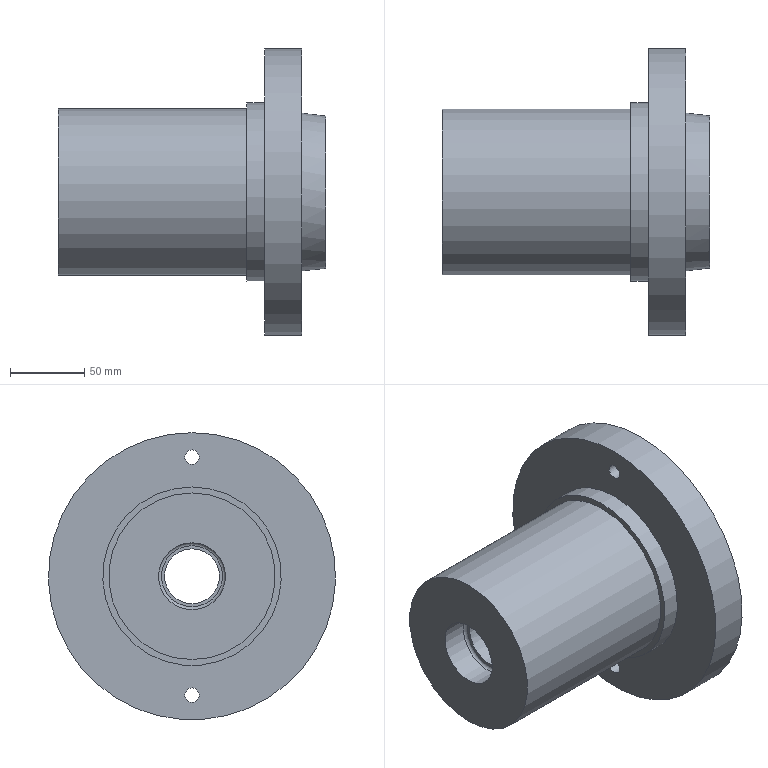Component | NX | CA614_SPINDLE | 1 solid | 16 faces | box 179.52 x 193 x 193 mm | volume 1954498 mm3 | cylinder 6 | plane 6 | cone 3 | torus 1 | commonest cylinder face diameters 9.732 x2 193 x1 45 x1 112 x1 120 x1
STEP:
#1=CARTESIAN_POINT('',(0.,0.,0.));
#2=DIRECTION('',(0.,0.,1.));
#3=DIRECTION('',(1.,0.,0.));
#4=AXIS2_PLACEMENT_3D('',#1,#2,#3);
#5=CARTESIAN_POINT('',(-50.,0.,96.5));
#6=VERTEX_POINT('',#5);
#7=CARTESIAN_POINT('',(-50.,0.,0.));
#8=DIRECTION('',(-1.,0.,0.));
#9=DIRECTION('',(0.,0.,1.));
#10=AXIS2_PLACEMENT_3D('',#7,#8,#9);
#11=CIRCLE('',#10,96.5);
#12=CARTESIAN_POINT('',(-34.,0.,0.));
#13=DIRECTION('',(-1.,0.,0.));
#14=DIRECTION('',(0.,0.,1.));
#15=AXIS2_PLACEMENT_3D('',#12,#13,#14);
#16=CYLINDRICAL_SURFACE('',#15,96.5);
#17=CARTESIAN_POINT('',(0.,16.));
#18=DIRECTION('',(1.,0.));
#19=VECTOR('',#18,1.);
#20=LINE('',#17,#19);
#21=(GEOMETRIC_REPRESENTATION_CONTEXT(2)PARAMETRIC_REPRESENTATION_CONTEXT()REPRESENTATION_CONTEXT('',''));
#22=DEFINITIONAL_REPRESENTATION('',(#20),#21);
#23=PCURVE('',#16,#22);
#24=CARTESIAN_POINT('',(-50.,96.5,0.));
#25=DIRECTION('',(1.,0.,0.));
#26=DIRECTION('',(0.,0.,-1.));
#27=AXIS2_PLACEMENT_3D('',#24,#25,#26);
#28=PLANE('',#27);
#29=CARTESIAN_POINT('',(-96.5,-96.5));
#30=CARTESIAN_POINT('',(-96.5,70.643));
#31=CARTESIAN_POINT('',(48.25,-12.929));
#32=CARTESIAN_POINT('',(193.,-96.5));
#33=CARTESIAN_POINT('',(48.25,-180.071));
#34=CARTESIAN_POINT('',(-96.5,-263.643));
#35=CARTESIAN_POINT('',(-96.5,-96.5));
#36=(BOUNDED_CURVE()B_SPLINE_CURVE(2,(#29,#30,#31,#32,#33,#34,#35),.UNSPECIFIED.,.T.,.F.)B_SPLINE_CURVE_WITH_KNOTS((1,2,2,2,2,1),(-2.094,0.,2.094,4.189,6.283,8.378),.UNSPECIFIED.)CURVE()GEOMETRIC_REPRESENTATION_ITEM()RATIONAL_B_SPLINE_CURVE((1.,0.5,1.,0.5,1.,0.5,1.))REPRESENTATION_ITEM(''));
#37=(GEOMETRIC_REPRESENTATION_CONTEXT(2)PARAMETRIC_REPRESENTATION_CONTEXT()REPRESENTATION_CONTEXT('',''));
#38=DEFINITIONAL_REPRESENTATION('',(#36),#37);
#39=PCURVE('',#28,#38);
#40=SURFACE_CURVE('',#11,(#23,#39),.PCURVE_S1.);
#41=EDGE_CURVE('',#6,#6,#40,.T.);
#42=ORIENTED_EDGE('',*,*,#41,.T.);
#43=CARTESIAN_POINT('',(-75.,0.,96.5));
#44=VERTEX_POINT('',#43);
#45=CARTESIAN_POINT('',(-50.,0.,96.5));
#46=CARTESIAN_POINT('',(-75.,0.,96.5));
#47=B_SPLINE_CURVE_WITH_KNOTS('',1,(#45,#46),.UNSPECIFIED.,.F.,.F.,(2,2),(16.,41.),.PIECEWISE_BEZIER_KNOTS.);
#48=CARTESIAN_POINT('',(6.283,0.));
#49=DIRECTION('',(0.,1.));
#50=VECTOR('',#49,1.);
#51=LINE('',#48,#50);
#52=(GEOMETRIC_REPRESENTATION_CONTEXT(2)PARAMETRIC_REPRESENTATION_CONTEXT()REPRESENTATION_CONTEXT('',''));
#53=DEFINITIONAL_REPRESENTATION('',(#51),#52);
#54=PCURVE('',#16,#53);
#55=CARTESIAN_POINT('',(0.,0.));
#56=DIRECTION('',(0.,1.));
#57=VECTOR('',#56,1.);
#58=LINE('',#55,#57);
#59=(GEOMETRIC_REPRESENTATION_CONTEXT(2)PARAMETRIC_REPRESENTATION_CONTEXT()REPRESENTATION_CONTEXT('',''));
#60=DEFINITIONAL_REPRESENTATION('',(#58),#59);
#61=PCURVE('',#16,#60);
#62=SEAM_CURVE('',#47,(#54,#61),.PCURVE_S1.);
#63=EDGE_CURVE('',#6,#44,#62,.T.);
#64=ORIENTED_EDGE('',*,*,#63,.T.);
#65=CARTESIAN_POINT('',(-75.,0.,0.));
#66=DIRECTION('',(-1.,0.,0.));
#67=DIRECTION('',(0.,0.,1.));
#68=AXIS2_PLACEMENT_3D('',#65,#66,#67);
#69=CIRCLE('',#68,96.5);
#70=CARTESIAN_POINT('',(0.,41.));
#71=DIRECTION('',(1.,0.));
#72=VECTOR('',#71,1.);
#73=LINE('',#70,#72);
#74=(GEOMETRIC_REPRESENTATION_CONTEXT(2)PARAMETRIC_REPRESENTATION_CONTEXT()REPRESENTATION_CONTEXT('',''));
#75=DEFINITIONAL_REPRESENTATION('',(#73),#74);
#76=PCURVE('',#16,#75);
#77=CARTESIAN_POINT('',(-75.,60.,0.));
#78=DIRECTION('',(-1.,0.,0.));
#79=DIRECTION('',(0.,0.,1.));
#80=AXIS2_PLACEMENT_3D('',#77,#78,#79);
#81=PLANE('',#80);
#82=CARTESIAN_POINT('',(0.,-60.));
#83=DIRECTION('',(1.,0.));
#84=AXIS2_PLACEMENT_2D('',#82,#83);
#85=CIRCLE('',#84,96.5);
#86=(GEOMETRIC_REPRESENTATION_CONTEXT(2)PARAMETRIC_REPRESENTATION_CONTEXT()REPRESENTATION_CONTEXT('',''));
#87=DEFINITIONAL_REPRESENTATION('',(#85),#86);
#88=PCURVE('',#81,#87);
#89=SURFACE_CURVE('',#69,(#76,#88),.PCURVE_S1.);
#90=EDGE_CURVE('',#44,#44,#89,.T.);
#91=ORIENTED_EDGE('',*,*,#90,.F.);
#92=ORIENTED_EDGE('',*,*,#63,.F.);
#93=EDGE_LOOP('',(#42,#64,#91,#92));
#94=FACE_BOUND('',#93,.T.);
#95=ADVANCED_FACE('',(#94),#16,.T.);
#96=CARTESIAN_POINT('',(-50.,0.,75.134));
#97=VERTEX_POINT('',#96);
#98=CARTESIAN_POINT('',(-50.,0.,80.));
#99=DIRECTION('',(1.,0.,0.));
#100=DIRECTION('',(0.,0.,-1.));
#101=AXIS2_PLACEMENT_3D('',#98,#99,#100);
#102=CIRCLE('',#101,4.866);
#103=CARTESIAN_POINT('',(-80.,-96.5));
#104=DIRECTION('',(1.,0.));
#105=AXIS2_PLACEMENT_2D('',#103,#104);
#106=CIRCLE('',#105,4.866);
#107=(GEOMETRIC_REPRESENTATION_CONTEXT(2)PARAMETRIC_REPRESENTATION_CONTEXT()REPRESENTATION_CONTEXT('',''));
#108=DEFINITIONAL_REPRESENTATION('',(#106),#107);
#109=PCURVE('',#28,#108);
#110=CARTESIAN_POINT('',(-75.,0.,80.));
#111=DIRECTION('',(1.,0.,0.));
#112=DIRECTION('',(0.,0.,-1.));
#113=AXIS2_PLACEMENT_3D('',#110,#111,#112);
#114=CYLINDRICAL_SURFACE('',#113,4.866);
#115=CARTESIAN_POINT('',(0.,25.));
#116=DIRECTION('',(1.,0.));
#117=VECTOR('',#116,1.);
#118=LINE('',#115,#117);
#119=(GEOMETRIC_REPRESENTATION_CONTEXT(2)PARAMETRIC_REPRESENTATION_CONTEXT()REPRESENTATION_CONTEXT('',''));
#120=DEFINITIONAL_REPRESENTATION('',(#118),#119);
#121=PCURVE('',#114,#120);
#122=SURFACE_CURVE('',#102,(#109,#121),.PCURVE_S1.);
#123=EDGE_CURVE('',#97,#97,#122,.T.);
#124=ORIENTED_EDGE('',*,*,#123,.F.);
#125=EDGE_LOOP('',(#124));
#126=FACE_BOUND('',#125,.T.);
#127=CARTESIAN_POINT('',(-50.,0.,-84.866));
#128=VERTEX_POINT('',#127);
#129=CARTESIAN_POINT('',(-50.,0.,-80.));
#130=DIRECTION('',(1.,0.,0.));
#131=DIRECTION('',(0.,0.,-1.));
#132=AXIS2_PLACEMENT_3D('',#129,#130,#131);
#133=CIRCLE('',#132,4.866);
#134=CARTESIAN_POINT('',(80.,-96.5));
#135=DIRECTION('',(1.,0.));
#136=AXIS2_PLACEMENT_2D('',#134,#135);
#137=CIRCLE('',#136,4.866);
#138=(GEOMETRIC_REPRESENTATION_CONTEXT(2)PARAMETRIC_REPRESENTATION_CONTEXT()REPRESENTATION_CONTEXT('',''));
#139=DEFINITIONAL_REPRESENTATION('',(#137),#138);
#140=PCURVE('',#28,#139);
#141=CARTESIAN_POINT('',(-75.,0.,-80.));
#142=DIRECTION('',(1.,0.,0.));
#143=DIRECTION('',(0.,0.,-1.));
#144=AXIS2_PLACEMENT_3D('',#141,#142,#143);
#145=CYLINDRICAL_SURFACE('',#144,4.866);
#146=CARTESIAN_POINT('',(0.,25.));
#147=DIRECTION('',(1.,0.));
#148=VECTOR('',#147,1.);
#149=LINE('',#146,#148);
#150=(GEOMETRIC_REPRESENTATION_CONTEXT(2)PARAMETRIC_REPRESENTATION_CONTEXT()REPRESENTATION_CONTEXT('',''));
#151=DEFINITIONAL_REPRESENTATION('',(#149),#150);
#152=PCURVE('',#145,#151);
#153=SURFACE_CURVE('',#133,(#140,#152),.PCURVE_S1.);
#154=EDGE_CURVE('',#128,#128,#153,.T.);
#155=ORIENTED_EDGE('',*,*,#154,.F.);
#156=EDGE_LOOP('',(#155));
#157=FACE_BOUND('',#156,.T.);
#158=CARTESIAN_POINT('',(-50.,0.,53.186));
#159=VERTEX_POINT('',#158);
#160=CARTESIAN_POINT('',(-50.,0.,0.));
#161=DIRECTION('',(-1.,0.,0.));
#162=DIRECTION('',(0.,0.,1.));
#163=AXIS2_PLACEMENT_3D('',#160,#161,#162);
#164=CIRCLE('',#163,53.186);
#165=CARTESIAN_POINT('',(-53.186,-96.5));
#166=CARTESIAN_POINT('',(-53.186,-4.378));
#167=CARTESIAN_POINT('',(26.593,-50.439));
#168=CARTESIAN_POINT('',(106.373,-96.5));
#169=CARTESIAN_POINT('',(26.593,-142.561));
#170=CARTESIAN_POINT('',(-53.186,-188.622));
#171=CARTESIAN_POINT('',(-53.186,-96.5));
#172=(BOUNDED_CURVE()B_SPLINE_CURVE(2,(#165,#166,#167,#168,#169,#170,#171),.UNSPECIFIED.,.T.,.F.)B_SPLINE_CURVE_WITH_KNOTS((1,2,2,2,2,1),(-2.094,0.,2.094,4.189,6.283,8.378),.UNSPECIFIED.)CURVE()GEOMETRIC_REPRESENTATION_ITEM()RATIONAL_B_SPLINE_CURVE((1.,0.5,1.,0.5,1.,0.5,1.))REPRESENTATION_ITEM(''));
#173=(GEOMETRIC_REPRESENTATION_CONTEXT(2)PARAMETRIC_REPRESENTATION_CONTEXT()REPRESENTATION_CONTEXT('',''));
#174=DEFINITIONAL_REPRESENTATION('',(#172),#173);
#175=PCURVE('',#28,#174);
#176=CARTESIAN_POINT('',(-50.,0.,0.));
#177=DIRECTION('',(-1.,0.,0.));
#178=DIRECTION('',(0.,0.,1.));
#179=AXIS2_PLACEMENT_3D('',#176,#177,#178);
#180=CONICAL_SURFACE('',#179,53.186,0.1244);
#181=CARTESIAN_POINT('',(0.,0.));
#182=DIRECTION('',(1.,0.));
#183=VECTOR('',#182,1.);
#184=LINE('',#181,#183);
#185=(GEOMETRIC_REPRESENTATION_CONTEXT(2)PARAMETRIC_REPRESENTATION_CONTEXT()REPRESENTATION_CONTEXT('',''));
#186=DEFINITIONAL_REPRESENTATION('',(#184),#185);
#187=PCURVE('',#180,#186);
#188=SURFACE_CURVE('',#164,(#175,#187),.PCURVE_S1.);
#189=EDGE_CURVE('',#159,#159,#188,.T.);
#190=ORIENTED_EDGE('',*,*,#189,.T.);
#191=EDGE_LOOP('',(#190));
#192=FACE_BOUND('',#191,.T.);
#193=ORIENTED_EDGE('',*,*,#41,.F.);
#194=EDGE_LOOP('',(#193));
#195=FACE_BOUND('',#194,.T.);
#196=ADVANCED_FACE('',(#126,#157,#192,#195),#28,.T.);
#197=CARTESIAN_POINT('',(-34.,0.,51.187));
#198=VERTEX_POINT('',#197);
#199=CARTESIAN_POINT('',(-34.,0.,0.));
#200=DIRECTION('',(-1.,0.,0.));
#201=DIRECTION('',(0.,0.,1.));
#202=AXIS2_PLACEMENT_3D('',#199,#200,#201);
#203=CIRCLE('',#202,51.187);
#204=CARTESIAN_POINT('',(0.,-16.));
#205=DIRECTION('',(1.,0.));
#206=VECTOR('',#205,1.);
#207=LINE('',#204,#206);
#208=(GEOMETRIC_REPRESENTATION_CONTEXT(2)PARAMETRIC_REPRESENTATION_CONTEXT()REPRESENTATION_CONTEXT('',''));
#209=DEFINITIONAL_REPRESENTATION('',(#207),#208);
#210=PCURVE('',#180,#209);
#211=CARTESIAN_POINT('',(-34.,51.187,0.));
#212=DIRECTION('',(1.,0.,0.));
#213=DIRECTION('',(0.,0.,-1.));
#214=AXIS2_PLACEMENT_3D('',#211,#212,#213);
#215=PLANE('',#214);
#216=CARTESIAN_POINT('',(-51.187,-51.187));
#217=CARTESIAN_POINT('',(-51.187,37.471));
#218=CARTESIAN_POINT('',(25.593,-6.858));
#219=CARTESIAN_POINT('',(102.373,-51.187));
#220=CARTESIAN_POINT('',(25.593,-95.515));
#221=CARTESIAN_POINT('',(-51.187,-139.844));
#222=CARTESIAN_POINT('',(-51.187,-51.187));
#223=(BOUNDED_CURVE()B_SPLINE_CURVE(2,(#216,#217,#218,#219,#220,#221,#222),.UNSPECIFIED.,.T.,.F.)B_SPLINE_CURVE_WITH_KNOTS((1,2,2,2,2,1),(-2.094,0.,2.094,4.189,6.283,8.378),.UNSPECIFIED.)CURVE()GEOMETRIC_REPRESENTATION_ITEM()RATIONAL_B_SPLINE_CURVE((1.,0.5,1.,0.5,1.,0.5,1.))REPRESENTATION_ITEM(''));
#224=(GEOMETRIC_REPRESENTATION_CONTEXT(2)PARAMETRIC_REPRESENTATION_CONTEXT()REPRESENTATION_CONTEXT('',''));
#225=DEFINITIONAL_REPRESENTATION('',(#223),#224);
#226=PCURVE('',#215,#225);
#227=SURFACE_CURVE('',#203,(#210,#226),.PCURVE_S1.);
#228=EDGE_CURVE('',#198,#198,#227,.T.);
#229=ORIENTED_EDGE('',*,*,#228,.T.);
#230=CARTESIAN_POINT('',(-34.,0.,51.187));
#231=CARTESIAN_POINT('',(-50.,0.,53.186));
#232=B_SPLINE_CURVE_WITH_KNOTS('',1,(#230,#231),.UNSPECIFIED.,.F.,.F.,(2,2),(-16.125,0.),.PIECEWISE_BEZIER_KNOTS.);
#233=CARTESIAN_POINT('',(6.283,0.));
#234=DIRECTION('',(0.,1.));
#235=VECTOR('',#234,1.);
#236=LINE('',#233,#235);
#237=(GEOMETRIC_REPRESENTATION_CONTEXT(2)PARAMETRIC_REPRESENTATION_CONTEXT()REPRESENTATION_CONTEXT('',''));
#238=DEFINITIONAL_REPRESENTATION('',(#236),#237);
#239=PCURVE('',#180,#238);
#240=CARTESIAN_POINT('',(0.,0.));
#241=DIRECTION('',(0.,1.));
#242=VECTOR('',#241,1.);
#243=LINE('',#240,#242);
#244=(GEOMETRIC_REPRESENTATION_CONTEXT(2)PARAMETRIC_REPRESENTATION_CONTEXT()REPRESENTATION_CONTEXT('',''));
#245=DEFINITIONAL_REPRESENTATION('',(#243),#244);
#246=PCURVE('',#180,#245);
#247=SEAM_CURVE('',#232,(#239,#246),.PCURVE_S1.);
#248=EDGE_CURVE('',#198,#159,#247,.T.);
#249=ORIENTED_EDGE('',*,*,#248,.T.);
#250=ORIENTED_EDGE('',*,*,#189,.F.);
#251=ORIENTED_EDGE('',*,*,#248,.F.);
#252=EDGE_LOOP('',(#229,#249,#250,#251));
#253=FACE_BOUND('',#252,.T.);
#254=ADVANCED_FACE('',(#253),#180,.T.);
#255=CARTESIAN_POINT('',(-34.,0.,28.406));
#256=VERTEX_POINT('',#255);
#257=CARTESIAN_POINT('',(-34.,0.,0.));
#258=DIRECTION('',(-1.,0.,0.));
#259=DIRECTION('',(0.,0.,1.));
#260=AXIS2_PLACEMENT_3D('',#257,#258,#259);
#261=CIRCLE('',#260,28.406);
#262=CARTESIAN_POINT('',(-28.406,-51.187));
#263=CARTESIAN_POINT('',(-28.406,-1.986));
#264=CARTESIAN_POINT('',(14.203,-26.586));
#265=CARTESIAN_POINT('',(56.812,-51.187));
#266=CARTESIAN_POINT('',(14.203,-75.787));
#267=CARTESIAN_POINT('',(-28.406,-100.387));
#268=CARTESIAN_POINT('',(-28.406,-51.187));
#269=(BOUNDED_CURVE()B_SPLINE_CURVE(2,(#262,#263,#264,#265,#266,#267,#268),.UNSPECIFIED.,.T.,.F.)B_SPLINE_CURVE_WITH_KNOTS((1,2,2,2,2,1),(-2.094,0.,2.094,4.189,6.283,8.378),.UNSPECIFIED.)CURVE()GEOMETRIC_REPRESENTATION_ITEM()RATIONAL_B_SPLINE_CURVE((1.,0.5,1.,0.5,1.,0.5,1.))REPRESENTATION_ITEM(''));
#270=(GEOMETRIC_REPRESENTATION_CONTEXT(2)PARAMETRIC_REPRESENTATION_CONTEXT()REPRESENTATION_CONTEXT('',''));
#271=DEFINITIONAL_REPRESENTATION('',(#269),#270);
#272=PCURVE('',#215,#271);
#273=CARTESIAN_POINT('',(-34.,0.,0.));
#274=DIRECTION('',(1.,0.,0.));
#275=DIRECTION('',(0.,0.,-1.));
#276=AXIS2_PLACEMENT_3D('',#273,#274,#275);
#277=CONICAL_SURFACE('',#276,28.406,0.5236);
#278=CARTESIAN_POINT('',(9.425,0.));
#279=DIRECTION('',(-1.,0.));
#280=VECTOR('',#279,1.);
#281=LINE('',#278,#280);
#282=(GEOMETRIC_REPRESENTATION_CONTEXT(2)PARAMETRIC_REPRESENTATION_CONTEXT()REPRESENTATION_CONTEXT('',''));
#283=DEFINITIONAL_REPRESENTATION('',(#281),#282);
#284=PCURVE('',#277,#283);
#285=SURFACE_CURVE('',#261,(#272,#284),.PCURVE_S1.);
#286=EDGE_CURVE('',#256,#256,#285,.T.);
#287=ORIENTED_EDGE('',*,*,#286,.T.);
#288=EDGE_LOOP('',(#287));
#289=FACE_BOUND('',#288,.T.);
#290=ORIENTED_EDGE('',*,*,#228,.F.);
#291=EDGE_LOOP('',(#290));
#292=FACE_BOUND('',#291,.T.);
#293=ADVANCED_FACE('',(#289,#292),#215,.T.);
#294=CARTESIAN_POINT('',(-37.,0.,26.674));
#295=VERTEX_POINT('',#294);
#296=CARTESIAN_POINT('',(-37.,0.,0.));
#297=DIRECTION('',(-1.,0.,0.));
#298=DIRECTION('',(0.,0.,1.));
#299=AXIS2_PLACEMENT_3D('',#296,#297,#298);
#300=CIRCLE('',#299,26.674);
#301=CARTESIAN_POINT('',(9.425,-3.));
#302=DIRECTION('',(-1.,0.));
#303=VECTOR('',#302,1.);
#304=LINE('',#301,#303);
#305=(GEOMETRIC_REPRESENTATION_CONTEXT(2)PARAMETRIC_REPRESENTATION_CONTEXT()REPRESENTATION_CONTEXT('',''));
#306=DEFINITIONAL_REPRESENTATION('',(#304),#305);
#307=PCURVE('',#277,#306);
#308=CARTESIAN_POINT('',(-37.,0.,0.));
#309=DIRECTION('',(1.,0.,0.));
#310=DIRECTION('',(0.,0.,-1.));
#311=AXIS2_PLACEMENT_3D('',#308,#309,#310);
#312=CONICAL_SURFACE('',#311,26.674,0.05213);
#313=CARTESIAN_POINT('',(9.425,0.));
#314=DIRECTION('',(-1.,0.));
#315=VECTOR('',#314,1.);
#316=LINE('',#313,#315);
#317=(GEOMETRIC_REPRESENTATION_CONTEXT(2)PARAMETRIC_REPRESENTATION_CONTEXT()REPRESENTATION_CONTEXT('',''));
#318=DEFINITIONAL_REPRESENTATION('',(#316),#317);
#319=PCURVE('',#312,#318);
#320=SURFACE_CURVE('',#300,(#307,#319),.PCURVE_S1.);
#321=EDGE_CURVE('',#295,#295,#320,.T.);
#322=ORIENTED_EDGE('',*,*,#321,.F.);
#323=CARTESIAN_POINT('',(-37.,0.,26.674));
#324=CARTESIAN_POINT('',(-34.,0.,28.406));
#325=B_SPLINE_CURVE_WITH_KNOTS('',1,(#323,#324),.UNSPECIFIED.,.F.,.F.,(2,2),(-3.464,0.),.PIECEWISE_BEZIER_KNOTS.);
#326=CARTESIAN_POINT('',(9.425,0.));
#327=DIRECTION('',(0.,1.));
#328=VECTOR('',#327,1.);
#329=LINE('',#326,#328);
#330=(GEOMETRIC_REPRESENTATION_CONTEXT(2)PARAMETRIC_REPRESENTATION_CONTEXT()REPRESENTATION_CONTEXT('',''));
#331=DEFINITIONAL_REPRESENTATION('',(#329),#330);
#332=PCURVE('',#277,#331);
#333=CARTESIAN_POINT('',(3.142,0.));
#334=DIRECTION('',(0.,1.));
#335=VECTOR('',#334,1.);
#336=LINE('',#333,#335);
#337=(GEOMETRIC_REPRESENTATION_CONTEXT(2)PARAMETRIC_REPRESENTATION_CONTEXT()REPRESENTATION_CONTEXT('',''));
#338=DEFINITIONAL_REPRESENTATION('',(#336),#337);
#339=PCURVE('',#277,#338);
#340=SEAM_CURVE('',#325,(#332,#339),.PCURVE_S1.);
#341=EDGE_CURVE('',#295,#256,#340,.T.);
#342=ORIENTED_EDGE('',*,*,#341,.T.);
#343=ORIENTED_EDGE('',*,*,#286,.T.);
#344=ORIENTED_EDGE('',*,*,#341,.F.);
#345=EDGE_LOOP('',(#322,#342,#343,#344));
#346=FACE_BOUND('',#345,.F.);
#347=ADVANCED_FACE('',(#346),#277,.F.);
#348=CARTESIAN_POINT('',(-194.,0.,18.483));
#349=VERTEX_POINT('',#348);
#350=CARTESIAN_POINT('',(-194.,0.,0.));
#351=DIRECTION('',(-1.,0.,0.));
#352=DIRECTION('',(0.,0.,1.));
#353=AXIS2_PLACEMENT_3D('',#350,#351,#352);
#354=CIRCLE('',#353,18.483);
#355=CARTESIAN_POINT('',(9.425,-157.));
#356=DIRECTION('',(-1.,0.));
#357=VECTOR('',#356,1.);
#358=LINE('',#355,#357);
#359=(GEOMETRIC_REPRESENTATION_CONTEXT(2)PARAMETRIC_REPRESENTATION_CONTEXT()REPRESENTATION_CONTEXT('',''));
#360=DEFINITIONAL_REPRESENTATION('',(#358),#359);
#361=PCURVE('',#312,#360);
#362=CARTESIAN_POINT('',(-194.,18.483,0.));
#363=DIRECTION('',(-1.,0.,0.));
#364=DIRECTION('',(0.,0.,1.));
#365=AXIS2_PLACEMENT_3D('',#362,#363,#364);
#366=PLANE('',#365);
#367=CARTESIAN_POINT('',(0.,-18.483));
#368=DIRECTION('',(1.,0.));
#369=AXIS2_PLACEMENT_2D('',#367,#368);
#370=CIRCLE('',#369,18.483);
#371=(GEOMETRIC_REPRESENTATION_CONTEXT(2)PARAMETRIC_REPRESENTATION_CONTEXT()REPRESENTATION_CONTEXT('',''));
#372=DEFINITIONAL_REPRESENTATION('',(#370),#371);
#373=PCURVE('',#366,#372);
#374=SURFACE_CURVE('',#354,(#361,#373),.PCURVE_S1.);
#375=EDGE_CURVE('',#349,#349,#374,.T.);
#376=ORIENTED_EDGE('',*,*,#375,.F.);
#377=CARTESIAN_POINT('',(-194.,0.,18.483));
#378=CARTESIAN_POINT('',(-37.,0.,26.674));
#379=B_SPLINE_CURVE_WITH_KNOTS('',1,(#377,#378),.UNSPECIFIED.,.F.,.F.,(2,2),(-157.214,0.),.PIECEWISE_BEZIER_KNOTS.);
#380=CARTESIAN_POINT('',(9.425,0.));
#381=DIRECTION('',(0.,1.));
#382=VECTOR('',#381,1.);
#383=LINE('',#380,#382);
#384=(GEOMETRIC_REPRESENTATION_CONTEXT(2)PARAMETRIC_REPRESENTATION_CONTEXT()REPRESENTATION_CONTEXT('',''));
#385=DEFINITIONAL_REPRESENTATION('',(#383),#384);
#386=PCURVE('',#312,#385);
#387=CARTESIAN_POINT('',(3.142,0.));
#388=DIRECTION('',(0.,1.));
#389=VECTOR('',#388,1.);
#390=LINE('',#387,#389);
#391=(GEOMETRIC_REPRESENTATION_CONTEXT(2)PARAMETRIC_REPRESENTATION_CONTEXT()REPRESENTATION_CONTEXT('',''));
#392=DEFINITIONAL_REPRESENTATION('',(#390),#391);
#393=PCURVE('',#312,#392);
#394=SEAM_CURVE('',#379,(#386,#393),.PCURVE_S1.);
#395=EDGE_CURVE('',#349,#295,#394,.T.);
#396=ORIENTED_EDGE('',*,*,#395,.T.);
#397=ORIENTED_EDGE('',*,*,#321,.T.);
#398=ORIENTED_EDGE('',*,*,#395,.F.);
#399=EDGE_LOOP('',(#376,#396,#397,#398));
#400=FACE_BOUND('',#399,.F.);
#401=ADVANCED_FACE('',(#400),#312,.F.);
#402=CARTESIAN_POINT('',(-194.,0.,20.5));
#403=VERTEX_POINT('',#402);
#404=CARTESIAN_POINT('',(-194.,0.,0.));
#405=DIRECTION('',(-1.,0.,0.));
#406=DIRECTION('',(0.,0.,1.));
#407=AXIS2_PLACEMENT_3D('',#404,#405,#406);
#408=CIRCLE('',#407,20.5);
#409=CARTESIAN_POINT('',(0.,-18.483));
#410=DIRECTION('',(1.,0.));
#411=AXIS2_PLACEMENT_2D('',#409,#410);
#412=CIRCLE('',#411,20.5);
#413=(GEOMETRIC_REPRESENTATION_CONTEXT(2)PARAMETRIC_REPRESENTATION_CONTEXT()REPRESENTATION_CONTEXT('',''));
#414=DEFINITIONAL_REPRESENTATION('',(#412),#413);
#415=PCURVE('',#366,#414);
#416=CARTESIAN_POINT('',(-196.,0.,0.));
#417=DIRECTION('',(-1.,0.,0.));
#418=DIRECTION('',(0.,0.,1.));
#419=AXIS2_PLACEMENT_3D('',#416,#417,#418);
#420=TOROIDAL_SURFACE('',#419,20.5,2.);
#421=CARTESIAN_POINT('',(0.,4.712));
#422=DIRECTION('',(1.,0.));
#423=VECTOR('',#422,1.);
#424=LINE('',#421,#423);
#425=(GEOMETRIC_REPRESENTATION_CONTEXT(2)PARAMETRIC_REPRESENTATION_CONTEXT()REPRESENTATION_CONTEXT('',''));
#426=DEFINITIONAL_REPRESENTATION('',(#424),#425);
#427=PCURVE('',#420,#426);
#428=SURFACE_CURVE('',#408,(#415,#427),.PCURVE_S1.);
#429=EDGE_CURVE('',#403,#403,#428,.T.);
#430=ORIENTED_EDGE('',*,*,#429,.T.);
#431=EDGE_LOOP('',(#430));
#432=FACE_BOUND('',#431,.T.);
#433=ORIENTED_EDGE('',*,*,#375,.F.);
#434=EDGE_LOOP('',(#433));
#435=FACE_BOUND('',#434,.T.);
#436=ADVANCED_FACE('',(#432,#435),#366,.T.);
#437=CARTESIAN_POINT('',(-196.,0.,22.5));
#438=VERTEX_POINT('',#437);
#439=CARTESIAN_POINT('',(-196.,0.,0.));
#440=DIRECTION('',(-1.,0.,0.));
#441=DIRECTION('',(0.,0.,1.));
#442=AXIS2_PLACEMENT_3D('',#439,#440,#441);
#443=CIRCLE('',#442,22.5);
#444=CARTESIAN_POINT('',(0.,6.283));
#445=DIRECTION('',(1.,0.));
#446=VECTOR('',#445,1.);
#447=LINE('',#444,#446);
#448=(GEOMETRIC_REPRESENTATION_CONTEXT(2)PARAMETRIC_REPRESENTATION_CONTEXT()REPRESENTATION_CONTEXT('',''));
#449=DEFINITIONAL_REPRESENTATION('',(#447),#448);
#450=PCURVE('',#420,#449);
#451=CARTESIAN_POINT('',(-34.,0.,0.));
#452=DIRECTION('',(-1.,0.,0.));
#453=DIRECTION('',(0.,0.,1.));
#454=AXIS2_PLACEMENT_3D('',#451,#452,#453);
#455=CYLINDRICAL_SURFACE('',#454,22.5);
#456=CARTESIAN_POINT('',(0.,162.));
#457=DIRECTION('',(1.,0.));
#458=VECTOR('',#457,1.);
#459=LINE('',#456,#458);
#460=(GEOMETRIC_REPRESENTATION_CONTEXT(2)PARAMETRIC_REPRESENTATION_CONTEXT()REPRESENTATION_CONTEXT('',''));
#461=DEFINITIONAL_REPRESENTATION('',(#459),#460);
#462=PCURVE('',#455,#461);
#463=SURFACE_CURVE('',#443,(#450,#462),.PCURVE_S1.);
#464=EDGE_CURVE('',#438,#438,#463,.T.);
#465=ORIENTED_EDGE('',*,*,#464,.F.);
#466=CARTESIAN_POINT('',(-194.,-0.,20.5));
#467=CARTESIAN_POINT('',(-194.,-0.,21.035));
#468=CARTESIAN_POINT('',(-194.17,-0.,21.555));
#469=CARTESIAN_POINT('',(-194.496,-0.,22.004));
#470=CARTESIAN_POINT('',(-194.945,-0.,22.33));
#471=CARTESIAN_POINT('',(-195.465,-0.,22.5));
#472=CARTESIAN_POINT('',(-196.,-0.,22.5));
#473=(BOUNDED_CURVE()B_SPLINE_CURVE(6,(#466,#467,#468,#469,#470,#471,#472),.UNSPECIFIED.,.F.,.F.)B_SPLINE_CURVE_WITH_KNOTS((7,7),(-1.571,0.),.PIECEWISE_BEZIER_KNOTS.)CURVE()GEOMETRIC_REPRESENTATION_ITEM()RATIONAL_B_SPLINE_CURVE((1.031,1.01,0.9979,0.994,0.9979,1.01,1.031))REPRESENTATION_ITEM(''));
#474=CARTESIAN_POINT('',(0.,6.283));
#475=DIRECTION('',(0.,1.));
#476=VECTOR('',#475,1.);
#477=LINE('',#474,#476);
#478=(GEOMETRIC_REPRESENTATION_CONTEXT(2)PARAMETRIC_REPRESENTATION_CONTEXT()REPRESENTATION_CONTEXT('',''));
#479=DEFINITIONAL_REPRESENTATION('',(#477),#478);
#480=PCURVE('',#420,#479);
#481=CARTESIAN_POINT('',(6.283,6.283));
#482=DIRECTION('',(0.,1.));
#483=VECTOR('',#482,1.);
#484=LINE('',#481,#483);
#485=(GEOMETRIC_REPRESENTATION_CONTEXT(2)PARAMETRIC_REPRESENTATION_CONTEXT()REPRESENTATION_CONTEXT('',''));
#486=DEFINITIONAL_REPRESENTATION('',(#484),#485);
#487=PCURVE('',#420,#486);
#488=SEAM_CURVE('',#473,(#480,#487),.PCURVE_S1.);
#489=EDGE_CURVE('',#403,#438,#488,.T.);
#490=ORIENTED_EDGE('',*,*,#489,.F.);
#491=ORIENTED_EDGE('',*,*,#429,.T.);
#492=ORIENTED_EDGE('',*,*,#489,.T.);
#493=EDGE_LOOP('',(#465,#490,#491,#492));
#494=FACE_BOUND('',#493,.F.);
#495=ADVANCED_FACE('',(#494),#420,.F.);
#496=CARTESIAN_POINT('',(-213.52,0.,22.5));
#497=VERTEX_POINT('',#496);
#498=CARTESIAN_POINT('',(-213.52,0.,0.));
#499=DIRECTION('',(-1.,0.,0.));
#500=DIRECTION('',(0.,0.,1.));
#501=AXIS2_PLACEMENT_3D('',#498,#499,#500);
#502=CIRCLE('',#501,22.5);
#503=CARTESIAN_POINT('',(0.,179.52));
#504=DIRECTION('',(1.,0.));
#505=VECTOR('',#504,1.);
#506=LINE('',#503,#505);
#507=(GEOMETRIC_REPRESENTATION_CONTEXT(2)PARAMETRIC_REPRESENTATION_CONTEXT()REPRESENTATION_CONTEXT('',''));
#508=DEFINITIONAL_REPRESENTATION('',(#506),#507);
#509=PCURVE('',#455,#508);
#510=CARTESIAN_POINT('',(-213.52,22.5,0.));
#511=DIRECTION('',(-1.,0.,0.));
#512=DIRECTION('',(0.,0.,1.));
#513=AXIS2_PLACEMENT_3D('',#510,#511,#512);
#514=PLANE('',#513);
#515=CARTESIAN_POINT('',(0.,-22.5));
#516=DIRECTION('',(1.,0.));
#517=AXIS2_PLACEMENT_2D('',#515,#516);
#518=CIRCLE('',#517,22.5);
#519=(GEOMETRIC_REPRESENTATION_CONTEXT(2)PARAMETRIC_REPRESENTATION_CONTEXT()REPRESENTATION_CONTEXT('',''));
#520=DEFINITIONAL_REPRESENTATION('',(#518),#519);
#521=PCURVE('',#514,#520);
#522=SURFACE_CURVE('',#502,(#509,#521),.PCURVE_S1.);
#523=EDGE_CURVE('',#497,#497,#522,.T.);
#524=ORIENTED_EDGE('',*,*,#523,.F.);
#525=CARTESIAN_POINT('',(-196.,-0.,22.5));
#526=CARTESIAN_POINT('',(-213.52,-0.,22.5));
#527=B_SPLINE_CURVE_WITH_KNOTS('',1,(#525,#526),.UNSPECIFIED.,.F.,.F.,(2,2),(162.,179.52),.PIECEWISE_BEZIER_KNOTS.);
#528=CARTESIAN_POINT('',(0.,0.));
#529=DIRECTION('',(0.,1.));
#530=VECTOR('',#529,1.);
#531=LINE('',#528,#530);
#532=(GEOMETRIC_REPRESENTATION_CONTEXT(2)PARAMETRIC_REPRESENTATION_CONTEXT()REPRESENTATION_CONTEXT('',''));
#533=DEFINITIONAL_REPRESENTATION('',(#531),#532);
#534=PCURVE('',#455,#533);
#535=CARTESIAN_POINT('',(6.283,0.));
#536=DIRECTION('',(0.,1.));
#537=VECTOR('',#536,1.);
#538=LINE('',#535,#537);
#539=(GEOMETRIC_REPRESENTATION_CONTEXT(2)PARAMETRIC_REPRESENTATION_CONTEXT()REPRESENTATION_CONTEXT('',''));
#540=DEFINITIONAL_REPRESENTATION('',(#538),#539);
#541=PCURVE('',#455,#540);
#542=SEAM_CURVE('',#527,(#534,#541),.PCURVE_S1.);
#543=EDGE_CURVE('',#438,#497,#542,.T.);
#544=ORIENTED_EDGE('',*,*,#543,.F.);
#545=ORIENTED_EDGE('',*,*,#464,.T.);
#546=ORIENTED_EDGE('',*,*,#543,.T.);
#547=EDGE_LOOP('',(#524,#544,#545,#546));
#548=FACE_BOUND('',#547,.F.);
#549=ADVANCED_FACE('',(#548),#455,.F.);
#550=CARTESIAN_POINT('',(-213.52,0.,56.));
#551=VERTEX_POINT('',#550);
#552=CARTESIAN_POINT('',(-213.52,0.,0.));
#553=DIRECTION('',(-1.,0.,0.));
#554=DIRECTION('',(0.,0.,1.));
#555=AXIS2_PLACEMENT_3D('',#552,#553,#554);
#556=CIRCLE('',#555,56.);
#557=CARTESIAN_POINT('',(0.,-22.5));
#558=DIRECTION('',(1.,0.));
#559=AXIS2_PLACEMENT_2D('',#557,#558);
#560=CIRCLE('',#559,56.);
#561=(GEOMETRIC_REPRESENTATION_CONTEXT(2)PARAMETRIC_REPRESENTATION_CONTEXT()REPRESENTATION_CONTEXT('',''));
#562=DEFINITIONAL_REPRESENTATION('',(#560),#561);
#563=PCURVE('',#514,#562);
#564=CARTESIAN_POINT('',(-34.,0.,0.));
#565=DIRECTION('',(-1.,0.,0.));
#566=DIRECTION('',(0.,0.,1.));
#567=AXIS2_PLACEMENT_3D('',#564,#565,#566);
#568=CYLINDRICAL_SURFACE('',#567,56.);
#569=CARTESIAN_POINT('',(0.,179.52));
#570=DIRECTION('',(1.,0.));
#571=VECTOR('',#570,1.);
#572=LINE('',#569,#571);
#573=(GEOMETRIC_REPRESENTATION_CONTEXT(2)PARAMETRIC_REPRESENTATION_CONTEXT()REPRESENTATION_CONTEXT('',''));
#574=DEFINITIONAL_REPRESENTATION('',(#572),#573);
#575=PCURVE('',#568,#574);
#576=SURFACE_CURVE('',#556,(#563,#575),.PCURVE_S1.);
#577=EDGE_CURVE('',#551,#551,#576,.T.);
#578=ORIENTED_EDGE('',*,*,#577,.T.);
#579=EDGE_LOOP('',(#578));
#580=FACE_BOUND('',#579,.T.);
#581=ORIENTED_EDGE('',*,*,#523,.F.);
#582=EDGE_LOOP('',(#581));
#583=FACE_BOUND('',#582,.T.);
#584=ADVANCED_FACE('',(#580,#583),#514,.T.);
#585=CARTESIAN_POINT('',(-87.,0.,56.));
#586=VERTEX_POINT('',#585);
#587=CARTESIAN_POINT('',(-87.,0.,0.));
#588=DIRECTION('',(-1.,0.,0.));
#589=DIRECTION('',(0.,0.,1.));
#590=AXIS2_PLACEMENT_3D('',#587,#588,#589);
#591=CIRCLE('',#590,56.);
#592=CARTESIAN_POINT('',(0.,53.));
#593=DIRECTION('',(1.,0.));
#594=VECTOR('',#593,1.);
#595=LINE('',#592,#594);
#596=(GEOMETRIC_REPRESENTATION_CONTEXT(2)PARAMETRIC_REPRESENTATION_CONTEXT()REPRESENTATION_CONTEXT('',''));
#597=DEFINITIONAL_REPRESENTATION('',(#595),#596);
#598=PCURVE('',#568,#597);
#599=CARTESIAN_POINT('',(-87.,56.,0.));
#600=DIRECTION('',(-1.,0.,0.));
#601=DIRECTION('',(0.,0.,1.));
#602=AXIS2_PLACEMENT_3D('',#599,#600,#601);
#603=PLANE('',#602);
#604=CARTESIAN_POINT('',(0.,-56.));
#605=DIRECTION('',(1.,0.));
#606=AXIS2_PLACEMENT_2D('',#604,#605);
#607=CIRCLE('',#606,56.);
#608=(GEOMETRIC_REPRESENTATION_CONTEXT(2)PARAMETRIC_REPRESENTATION_CONTEXT()REPRESENTATION_CONTEXT('',''));
#609=DEFINITIONAL_REPRESENTATION('',(#607),#608);
#610=PCURVE('',#603,#609);
#611=SURFACE_CURVE('',#591,(#598,#610),.PCURVE_S1.);
#612=EDGE_CURVE('',#586,#586,#611,.T.);
#613=ORIENTED_EDGE('',*,*,#612,.T.);
#614=CARTESIAN_POINT('',(-87.,0.,56.));
#615=CARTESIAN_POINT('',(-213.52,0.,56.));
#616=B_SPLINE_CURVE_WITH_KNOTS('',1,(#614,#615),.UNSPECIFIED.,.F.,.F.,(2,2),(53.,179.52),.PIECEWISE_BEZIER_KNOTS.);
#617=CARTESIAN_POINT('',(6.283,0.));
#618=DIRECTION('',(0.,1.));
#619=VECTOR('',#618,1.);
#620=LINE('',#617,#619);
#621=(GEOMETRIC_REPRESENTATION_CONTEXT(2)PARAMETRIC_REPRESENTATION_CONTEXT()REPRESENTATION_CONTEXT('',''));
#622=DEFINITIONAL_REPRESENTATION('',(#620),#621);
#623=PCURVE('',#568,#622);
#624=CARTESIAN_POINT('',(0.,0.));
#625=DIRECTION('',(0.,1.));
#626=VECTOR('',#625,1.);
#627=LINE('',#624,#626);
#628=(GEOMETRIC_REPRESENTATION_CONTEXT(2)PARAMETRIC_REPRESENTATION_CONTEXT()REPRESENTATION_CONTEXT('',''));
#629=DEFINITIONAL_REPRESENTATION('',(#627),#628);
#630=PCURVE('',#568,#629);
#631=SEAM_CURVE('',#616,(#623,#630),.PCURVE_S1.);
#632=EDGE_CURVE('',#586,#551,#631,.T.);
#633=ORIENTED_EDGE('',*,*,#632,.T.);
#634=ORIENTED_EDGE('',*,*,#577,.F.);
#635=ORIENTED_EDGE('',*,*,#632,.F.);
#636=EDGE_LOOP('',(#613,#633,#634,#635));
#637=FACE_BOUND('',#636,.T.);
#638=ADVANCED_FACE('',(#637),#568,.T.);
#639=CARTESIAN_POINT('',(-87.,0.,60.));
#640=VERTEX_POINT('',#639);
#641=CARTESIAN_POINT('',(-87.,0.,0.));
#642=DIRECTION('',(-1.,0.,0.));
#643=DIRECTION('',(0.,0.,1.));
#644=AXIS2_PLACEMENT_3D('',#641,#642,#643);
#645=CIRCLE('',#644,60.);
#646=CARTESIAN_POINT('',(0.,-56.));
#647=DIRECTION('',(1.,0.));
#648=AXIS2_PLACEMENT_2D('',#646,#647);
#649=CIRCLE('',#648,60.);
#650=(GEOMETRIC_REPRESENTATION_CONTEXT(2)PARAMETRIC_REPRESENTATION_CONTEXT()REPRESENTATION_CONTEXT('',''));
#651=DEFINITIONAL_REPRESENTATION('',(#649),#650);
#652=PCURVE('',#603,#651);
#653=CARTESIAN_POINT('',(-34.,0.,0.));
#654=DIRECTION('',(-1.,0.,0.));
#655=DIRECTION('',(0.,0.,1.));
#656=AXIS2_PLACEMENT_3D('',#653,#654,#655);
#657=CYLINDRICAL_SURFACE('',#656,60.);
#658=CARTESIAN_POINT('',(0.,53.));
#659=DIRECTION('',(1.,0.));
#660=VECTOR('',#659,1.);
#661=LINE('',#658,#660);
#662=(GEOMETRIC_REPRESENTATION_CONTEXT(2)PARAMETRIC_REPRESENTATION_CONTEXT()REPRESENTATION_CONTEXT('',''));
#663=DEFINITIONAL_REPRESENTATION('',(#661),#662);
#664=PCURVE('',#657,#663);
#665=SURFACE_CURVE('',#645,(#652,#664),.PCURVE_S1.);
#666=EDGE_CURVE('',#640,#640,#665,.T.);
#667=ORIENTED_EDGE('',*,*,#666,.T.);
#668=EDGE_LOOP('',(#667));
#669=FACE_BOUND('',#668,.T.);
#670=ORIENTED_EDGE('',*,*,#612,.F.);
#671=EDGE_LOOP('',(#670));
#672=FACE_BOUND('',#671,.T.);
#673=ADVANCED_FACE('',(#669,#672),#603,.T.);
#674=CARTESIAN_POINT('',(-75.,0.,60.));
#675=VERTEX_POINT('',#674);
#676=CARTESIAN_POINT('',(-75.,0.,0.));
#677=DIRECTION('',(-1.,0.,0.));
#678=DIRECTION('',(0.,0.,1.));
#679=AXIS2_PLACEMENT_3D('',#676,#677,#678);
#680=CIRCLE('',#679,60.);
#681=CARTESIAN_POINT('',(0.,41.));
#682=DIRECTION('',(1.,0.));
#683=VECTOR('',#682,1.);
#684=LINE('',#681,#683);
#685=(GEOMETRIC_REPRESENTATION_CONTEXT(2)PARAMETRIC_REPRESENTATION_CONTEXT()REPRESENTATION_CONTEXT('',''));
#686=DEFINITIONAL_REPRESENTATION('',(#684),#685);
#687=PCURVE('',#657,#686);
#688=CARTESIAN_POINT('',(0.,-60.));
#689=DIRECTION('',(1.,0.));
#690=AXIS2_PLACEMENT_2D('',#688,#689);
#691=CIRCLE('',#690,60.);
#692=(GEOMETRIC_REPRESENTATION_CONTEXT(2)PARAMETRIC_REPRESENTATION_CONTEXT()REPRESENTATION_CONTEXT('',''));
#693=DEFINITIONAL_REPRESENTATION('',(#691),#692);
#694=PCURVE('',#81,#693);
#695=SURFACE_CURVE('',#680,(#687,#694),.PCURVE_S1.);
#696=EDGE_CURVE('',#675,#675,#695,.T.);
#697=ORIENTED_EDGE('',*,*,#696,.T.);
#698=CARTESIAN_POINT('',(-75.,0.,60.));
#699=CARTESIAN_POINT('',(-87.,0.,60.));
#700=B_SPLINE_CURVE_WITH_KNOTS('',1,(#698,#699),.UNSPECIFIED.,.F.,.F.,(2,2),(41.,53.),.PIECEWISE_BEZIER_KNOTS.);
#701=CARTESIAN_POINT('',(6.283,0.));
#702=DIRECTION('',(0.,1.));
#703=VECTOR('',#702,1.);
#704=LINE('',#701,#703);
#705=(GEOMETRIC_REPRESENTATION_CONTEXT(2)PARAMETRIC_REPRESENTATION_CONTEXT()REPRESENTATION_CONTEXT('',''));
#706=DEFINITIONAL_REPRESENTATION('',(#704),#705);
#707=PCURVE('',#657,#706);
#708=CARTESIAN_POINT('',(0.,0.));
#709=DIRECTION('',(0.,1.));
#710=VECTOR('',#709,1.);
#711=LINE('',#708,#710);
#712=(GEOMETRIC_REPRESENTATION_CONTEXT(2)PARAMETRIC_REPRESENTATION_CONTEXT()REPRESENTATION_CONTEXT('',''));
#713=DEFINITIONAL_REPRESENTATION('',(#711),#712);
#714=PCURVE('',#657,#713);
#715=SEAM_CURVE('',#700,(#707,#714),.PCURVE_S1.);
#716=EDGE_CURVE('',#675,#640,#715,.T.);
#717=ORIENTED_EDGE('',*,*,#716,.T.);
#718=ORIENTED_EDGE('',*,*,#666,.F.);
#719=ORIENTED_EDGE('',*,*,#716,.F.);
#720=EDGE_LOOP('',(#697,#717,#718,#719));
#721=FACE_BOUND('',#720,.T.);
#722=ADVANCED_FACE('',(#721),#657,.T.);
#723=CARTESIAN_POINT('',(-75.,0.,84.866));
#724=VERTEX_POINT('',#723);
#725=CARTESIAN_POINT('',(-75.,-0.,75.134));
#726=VERTEX_POINT('',#725);
#727=CARTESIAN_POINT('',(-75.,0.,80.));
#728=DIRECTION('',(1.,0.,0.));
#729=DIRECTION('',(0.,0.,1.));
#730=AXIS2_PLACEMENT_3D('',#727,#728,#729);
#731=CIRCLE('',#730,4.866);
#732=CARTESIAN_POINT('',(84.866,-60.));
#733=CARTESIAN_POINT('',(84.866,-68.428));
#734=CARTESIAN_POINT('',(77.567,-64.214));
#735=CARTESIAN_POINT('',(70.268,-60.));
#736=CARTESIAN_POINT('',(77.567,-55.786));
#737=CARTESIAN_POINT('',(84.866,-51.572));
#738=CARTESIAN_POINT('',(84.866,-60.));
#739=(BOUNDED_CURVE()B_SPLINE_CURVE(2,(#732,#733,#734,#735,#736,#737,#738),.UNSPECIFIED.,.T.,.F.)B_SPLINE_CURVE_WITH_KNOTS((1,2,2,2,2,1),(-2.094,0.,2.094,4.189,6.283,8.378),.UNSPECIFIED.)CURVE()GEOMETRIC_REPRESENTATION_ITEM()RATIONAL_B_SPLINE_CURVE((1.,0.5,1.,0.5,1.,0.5,1.))REPRESENTATION_ITEM(''));
#740=(GEOMETRIC_REPRESENTATION_CONTEXT(2)PARAMETRIC_REPRESENTATION_CONTEXT()REPRESENTATION_CONTEXT('',''));
#741=DEFINITIONAL_REPRESENTATION('',(#739),#740);
#742=PCURVE('',#81,#741);
#743=CARTESIAN_POINT('',(3.142,0.));
#744=DIRECTION('',(1.,0.));
#745=VECTOR('',#744,1.);
#746=LINE('',#743,#745);
#747=(GEOMETRIC_REPRESENTATION_CONTEXT(2)PARAMETRIC_REPRESENTATION_CONTEXT()REPRESENTATION_CONTEXT('',''));
#748=DEFINITIONAL_REPRESENTATION('',(#746),#747);
#749=PCURVE('',#114,#748);
#750=SURFACE_CURVE('',#731,(#742,#749),.PCURVE_S1.);
#751=EDGE_CURVE('',#724,#726,#750,.T.);
#752=ORIENTED_EDGE('',*,*,#751,.T.);
#753=CARTESIAN_POINT('',(-75.,0.,80.));
#754=DIRECTION('',(1.,0.,0.));
#755=DIRECTION('',(0.,0.,1.));
#756=AXIS2_PLACEMENT_3D('',#753,#754,#755);
#757=CIRCLE('',#756,4.866);
#758=CARTESIAN_POINT('',(84.866,-60.));
#759=CARTESIAN_POINT('',(84.866,-68.428));
#760=CARTESIAN_POINT('',(77.567,-64.214));
#761=CARTESIAN_POINT('',(70.268,-60.));
#762=CARTESIAN_POINT('',(77.567,-55.786));
#763=CARTESIAN_POINT('',(84.866,-51.572));
#764=CARTESIAN_POINT('',(84.866,-60.));
#765=(BOUNDED_CURVE()B_SPLINE_CURVE(2,(#758,#759,#760,#761,#762,#763,#764),.UNSPECIFIED.,.T.,.F.)B_SPLINE_CURVE_WITH_KNOTS((1,2,2,2,2,1),(-2.094,0.,2.094,4.189,6.283,8.378),.UNSPECIFIED.)CURVE()GEOMETRIC_REPRESENTATION_ITEM()RATIONAL_B_SPLINE_CURVE((1.,0.5,1.,0.5,1.,0.5,1.))REPRESENTATION_ITEM(''));
#766=(GEOMETRIC_REPRESENTATION_CONTEXT(2)PARAMETRIC_REPRESENTATION_CONTEXT()REPRESENTATION_CONTEXT('',''));
#767=DEFINITIONAL_REPRESENTATION('',(#765),#766);
#768=PCURVE('',#81,#767);
#769=CARTESIAN_POINT('',(-3.142,0.));
#770=DIRECTION('',(1.,0.));
#771=VECTOR('',#770,1.);
#772=LINE('',#769,#771);
#773=(GEOMETRIC_REPRESENTATION_CONTEXT(2)PARAMETRIC_REPRESENTATION_CONTEXT()REPRESENTATION_CONTEXT('',''));
#774=DEFINITIONAL_REPRESENTATION('',(#772),#773);
#775=PCURVE('',#114,#774);
#776=SURFACE_CURVE('',#757,(#768,#775),.PCURVE_S1.);
#777=EDGE_CURVE('',#726,#724,#776,.T.);
#778=ORIENTED_EDGE('',*,*,#777,.T.);
#779=EDGE_LOOP('',(#752,#778));
#780=FACE_BOUND('',#779,.T.);
#781=CARTESIAN_POINT('',(-75.,0.,-75.134));
#782=VERTEX_POINT('',#781);
#783=CARTESIAN_POINT('',(-75.,-0.,-84.866));
#784=VERTEX_POINT('',#783);
#785=CARTESIAN_POINT('',(-75.,0.,-80.));
#786=DIRECTION('',(1.,0.,0.));
#787=DIRECTION('',(0.,0.,1.));
#788=AXIS2_PLACEMENT_3D('',#785,#786,#787);
#789=CIRCLE('',#788,4.866);
#790=CARTESIAN_POINT('',(-75.134,-60.));
#791=CARTESIAN_POINT('',(-75.134,-68.428));
#792=CARTESIAN_POINT('',(-82.433,-64.214));
#793=CARTESIAN_POINT('',(-89.732,-60.));
#794=CARTESIAN_POINT('',(-82.433,-55.786));
#795=CARTESIAN_POINT('',(-75.134,-51.572));
#796=CARTESIAN_POINT('',(-75.134,-60.));
#797=(BOUNDED_CURVE()B_SPLINE_CURVE(2,(#790,#791,#792,#793,#794,#795,#796),.UNSPECIFIED.,.T.,.F.)B_SPLINE_CURVE_WITH_KNOTS((1,2,2,2,2,1),(-2.094,0.,2.094,4.189,6.283,8.378),.UNSPECIFIED.)CURVE()GEOMETRIC_REPRESENTATION_ITEM()RATIONAL_B_SPLINE_CURVE((1.,0.5,1.,0.5,1.,0.5,1.))REPRESENTATION_ITEM(''));
#798=(GEOMETRIC_REPRESENTATION_CONTEXT(2)PARAMETRIC_REPRESENTATION_CONTEXT()REPRESENTATION_CONTEXT('',''));
#799=DEFINITIONAL_REPRESENTATION('',(#797),#798);
#800=PCURVE('',#81,#799);
#801=CARTESIAN_POINT('',(3.142,0.));
#802=DIRECTION('',(1.,0.));
#803=VECTOR('',#802,1.);
#804=LINE('',#801,#803);
#805=(GEOMETRIC_REPRESENTATION_CONTEXT(2)PARAMETRIC_REPRESENTATION_CONTEXT()REPRESENTATION_CONTEXT('',''));
#806=DEFINITIONAL_REPRESENTATION('',(#804),#805);
#807=PCURVE('',#145,#806);
#808=SURFACE_CURVE('',#789,(#800,#807),.PCURVE_S1.);
#809=EDGE_CURVE('',#782,#784,#808,.T.);
#810=ORIENTED_EDGE('',*,*,#809,.T.);
#811=CARTESIAN_POINT('',(-75.,0.,-80.));
#812=DIRECTION('',(1.,0.,0.));
#813=DIRECTION('',(0.,0.,1.));
#814=AXIS2_PLACEMENT_3D('',#811,#812,#813);
#815=CIRCLE('',#814,4.866);
#816=CARTESIAN_POINT('',(-75.134,-60.));
#817=CARTESIAN_POINT('',(-75.134,-68.428));
#818=CARTESIAN_POINT('',(-82.433,-64.214));
#819=CARTESIAN_POINT('',(-89.732,-60.));
#820=CARTESIAN_POINT('',(-82.433,-55.786));
#821=CARTESIAN_POINT('',(-75.134,-51.572));
#822=CARTESIAN_POINT('',(-75.134,-60.));
#823=(BOUNDED_CURVE()B_SPLINE_CURVE(2,(#816,#817,#818,#819,#820,#821,#822),.UNSPECIFIED.,.T.,.F.)B_SPLINE_CURVE_WITH_KNOTS((1,2,2,2,2,1),(-2.094,0.,2.094,4.189,6.283,8.378),.UNSPECIFIED.)CURVE()GEOMETRIC_REPRESENTATION_ITEM()RATIONAL_B_SPLINE_CURVE((1.,0.5,1.,0.5,1.,0.5,1.))REPRESENTATION_ITEM(''));
#824=(GEOMETRIC_REPRESENTATION_CONTEXT(2)PARAMETRIC_REPRESENTATION_CONTEXT()REPRESENTATION_CONTEXT('',''));
#825=DEFINITIONAL_REPRESENTATION('',(#823),#824);
#826=PCURVE('',#81,#825);
#827=CARTESIAN_POINT('',(-3.142,0.));
#828=DIRECTION('',(1.,0.));
#829=VECTOR('',#828,1.);
#830=LINE('',#827,#829);
#831=(GEOMETRIC_REPRESENTATION_CONTEXT(2)PARAMETRIC_REPRESENTATION_CONTEXT()REPRESENTATION_CONTEXT('',''));
#832=DEFINITIONAL_REPRESENTATION('',(#830),#831);
#833=PCURVE('',#145,#832);
#834=SURFACE_CURVE('',#815,(#826,#833),.PCURVE_S1.);
#835=EDGE_CURVE('',#784,#782,#834,.T.);
#836=ORIENTED_EDGE('',*,*,#835,.T.);
#837=EDGE_LOOP('',(#810,#836));
#838=FACE_BOUND('',#837,.T.);
#839=ORIENTED_EDGE('',*,*,#90,.T.);
#840=EDGE_LOOP('',(#839));
#841=FACE_BOUND('',#840,.T.);
#842=ORIENTED_EDGE('',*,*,#696,.F.);
#843=EDGE_LOOP('',(#842));
#844=FACE_BOUND('',#843,.T.);
#845=ADVANCED_FACE('',(#780,#838,#841,#844),#81,.T.);
#846=ORIENTED_EDGE('',*,*,#154,.F.);
#847=CARTESIAN_POINT('',(-75.,-0.,-84.866));
#848=CARTESIAN_POINT('',(-50.,-0.,-84.866));
#849=B_SPLINE_CURVE_WITH_KNOTS('',1,(#847,#848),.UNSPECIFIED.,.F.,.F.,(2,2),(0.,25.),.PIECEWISE_BEZIER_KNOTS.);
#850=CARTESIAN_POINT('',(0.,0.));
#851=DIRECTION('',(0.,1.));
#852=VECTOR('',#851,1.);
#853=LINE('',#850,#852);
#854=(GEOMETRIC_REPRESENTATION_CONTEXT(2)PARAMETRIC_REPRESENTATION_CONTEXT()REPRESENTATION_CONTEXT('',''));
#855=DEFINITIONAL_REPRESENTATION('',(#853),#854);
#856=PCURVE('',#145,#855);
#857=CARTESIAN_POINT('',(6.283,0.));
#858=DIRECTION('',(0.,1.));
#859=VECTOR('',#858,1.);
#860=LINE('',#857,#859);
#861=(GEOMETRIC_REPRESENTATION_CONTEXT(2)PARAMETRIC_REPRESENTATION_CONTEXT()REPRESENTATION_CONTEXT('',''));
#862=DEFINITIONAL_REPRESENTATION('',(#860),#861);
#863=PCURVE('',#145,#862);
#864=SEAM_CURVE('',#849,(#856,#863),.PCURVE_S1.);
#865=EDGE_CURVE('',#784,#128,#864,.T.);
#866=ORIENTED_EDGE('',*,*,#865,.F.);
#867=ORIENTED_EDGE('',*,*,#835,.T.);
#868=ORIENTED_EDGE('',*,*,#809,.T.);
#869=ORIENTED_EDGE('',*,*,#865,.T.);
#870=EDGE_LOOP('',(#846,#866,#867,#868,#869));
#871=FACE_BOUND('',#870,.F.);
#872=ADVANCED_FACE('',(#871),#145,.F.);
#873=ORIENTED_EDGE('',*,*,#123,.F.);
#874=CARTESIAN_POINT('',(-75.,-0.,75.134));
#875=CARTESIAN_POINT('',(-50.,-0.,75.134));
#876=B_SPLINE_CURVE_WITH_KNOTS('',1,(#874,#875),.UNSPECIFIED.,.F.,.F.,(2,2),(0.,25.),.PIECEWISE_BEZIER_KNOTS.);
#877=CARTESIAN_POINT('',(0.,0.));
#878=DIRECTION('',(0.,1.));
#879=VECTOR('',#878,1.);
#880=LINE('',#877,#879);
#881=(GEOMETRIC_REPRESENTATION_CONTEXT(2)PARAMETRIC_REPRESENTATION_CONTEXT()REPRESENTATION_CONTEXT('',''));
#882=DEFINITIONAL_REPRESENTATION('',(#880),#881);
#883=PCURVE('',#114,#882);
#884=CARTESIAN_POINT('',(6.283,0.));
#885=DIRECTION('',(0.,1.));
#886=VECTOR('',#885,1.);
#887=LINE('',#884,#886);
#888=(GEOMETRIC_REPRESENTATION_CONTEXT(2)PARAMETRIC_REPRESENTATION_CONTEXT()REPRESENTATION_CONTEXT('',''));
#889=DEFINITIONAL_REPRESENTATION('',(#887),#888);
#890=PCURVE('',#114,#889);
#891=SEAM_CURVE('',#876,(#883,#890),.PCURVE_S1.);
#892=EDGE_CURVE('',#726,#97,#891,.T.);
#893=ORIENTED_EDGE('',*,*,#892,.F.);
#894=ORIENTED_EDGE('',*,*,#777,.T.);
#895=ORIENTED_EDGE('',*,*,#751,.T.);
#896=ORIENTED_EDGE('',*,*,#892,.T.);
#897=EDGE_LOOP('',(#873,#893,#894,#895,#896));
#898=FACE_BOUND('',#897,.F.);
#899=ADVANCED_FACE('',(#898),#114,.F.);
#900=CLOSED_SHELL('',(#95,#196,#254,#293,#347,#401,#436,#495,#549,#584,#638,#673,#722,#845,#872,#899));
#901=MANIFOLD_SOLID_BREP('',#900);
#902=(LENGTH_UNIT()NAMED_UNIT(*)SI_UNIT(.MILLI.,.METRE.));
#903=UNCERTAINTY_MEASURE_WITH_UNIT(LENGTH_MEASURE(0.00001),#902,'','');
#904=(NAMED_UNIT(*)PLANE_ANGLE_UNIT()SI_UNIT($,.RADIAN.));
#905=(NAMED_UNIT(*)SI_UNIT($,.STERADIAN.)SOLID_ANGLE_UNIT());
#906=(GEOMETRIC_REPRESENTATION_CONTEXT(3)GLOBAL_UNCERTAINTY_ASSIGNED_CONTEXT((#903))GLOBAL_UNIT_ASSIGNED_CONTEXT((#902,#904,#905))REPRESENTATION_CONTEXT('',''));
#907=ADVANCED_BREP_SHAPE_REPRESENTATION('',(#4,#901),#906);